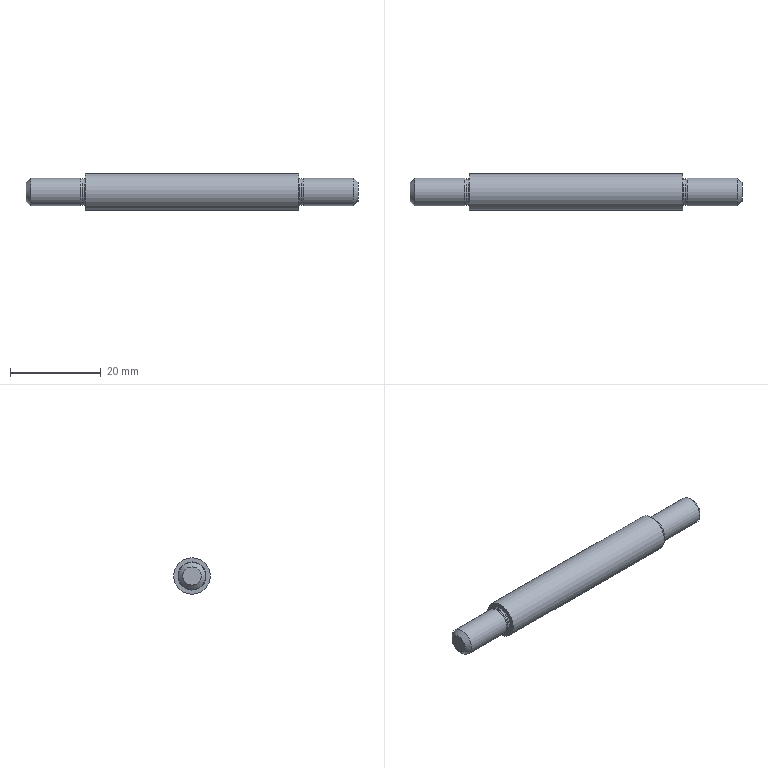Component | NX | SLIDING_GUIDE | 1 solid | 17 faces | box 73 x 8 x 8 mm | volume 3078 mm3 | cylinder 5 | plane 4 | cone 4 | torus 4 | commonest cylinder face diameters 6 x2 5.8 x2 8 x1
STEP:
#1=CARTESIAN_POINT('',(0.,0.,0.));
#2=DIRECTION('',(0.,0.,1.));
#3=DIRECTION('',(1.,0.,0.));
#4=AXIS2_PLACEMENT_3D('',#1,#2,#3);
#5=CARTESIAN_POINT('',(-36.5,15.,16.));
#6=VERTEX_POINT('',#5);
#7=CARTESIAN_POINT('',(-36.5,15.,18.));
#8=DIRECTION('',(-1.,0.,0.));
#9=DIRECTION('',(0.,0.,-1.));
#10=AXIS2_PLACEMENT_3D('',#7,#8,#9);
#11=CIRCLE('',#10,2.);
#12=CARTESIAN_POINT('',(-36.5,15.,21.));
#13=DIRECTION('',(1.,0.,0.));
#14=DIRECTION('',(0.,0.,-1.));
#15=AXIS2_PLACEMENT_3D('',#12,#13,#14);
#16=PLANE('',#15);
#17=CARTESIAN_POINT('',(5.,0.));
#18=CARTESIAN_POINT('',(5.,-3.464));
#19=CARTESIAN_POINT('',(2.,-1.732));
#20=CARTESIAN_POINT('',(-1.,-0.));
#21=CARTESIAN_POINT('',(2.,1.732));
#22=CARTESIAN_POINT('',(5.,3.464));
#23=CARTESIAN_POINT('',(5.,0.));
#24=(BOUNDED_CURVE()B_SPLINE_CURVE(2,(#17,#18,#19,#20,#21,#22,#23),.UNSPECIFIED.,.T.,.F.)B_SPLINE_CURVE_WITH_KNOTS((1,2,2,2,2,1),(-2.094,0.,2.094,4.189,6.283,8.378),.UNSPECIFIED.)CURVE()GEOMETRIC_REPRESENTATION_ITEM()RATIONAL_B_SPLINE_CURVE((1.,0.5,1.,0.5,1.,0.5,1.))REPRESENTATION_ITEM(''));
#25=(GEOMETRIC_REPRESENTATION_CONTEXT(2)PARAMETRIC_REPRESENTATION_CONTEXT()REPRESENTATION_CONTEXT('',''));
#26=DEFINITIONAL_REPRESENTATION('',(#24),#25);
#27=PCURVE('',#16,#26);
#28=CARTESIAN_POINT('',(-36.5,15.,18.));
#29=DIRECTION('',(1.,0.,0.));
#30=DIRECTION('',(0.,0.,-1.));
#31=AXIS2_PLACEMENT_3D('',#28,#29,#30);
#32=CONICAL_SURFACE('',#31,2.,0.7854);
#33=CARTESIAN_POINT('',(6.283,0.));
#34=DIRECTION('',(-1.,0.));
#35=VECTOR('',#34,1.);
#36=LINE('',#33,#35);
#37=(GEOMETRIC_REPRESENTATION_CONTEXT(2)PARAMETRIC_REPRESENTATION_CONTEXT()REPRESENTATION_CONTEXT('',''));
#38=DEFINITIONAL_REPRESENTATION('',(#36),#37);
#39=PCURVE('',#32,#38);
#40=SURFACE_CURVE('',#11,(#27,#39),.PCURVE_S1.);
#41=EDGE_CURVE('',#6,#6,#40,.T.);
#42=ORIENTED_EDGE('',*,*,#41,.T.);
#43=EDGE_LOOP('',(#42));
#44=FACE_BOUND('',#43,.T.);
#45=ADVANCED_FACE('',(#44),#16,.F.);
#46=CARTESIAN_POINT('',(-35.5,15.,15.));
#47=VERTEX_POINT('',#46);
#48=CARTESIAN_POINT('',(-35.5,15.,21.));
#49=VERTEX_POINT('',#48);
#50=CARTESIAN_POINT('',(-35.5,15.,18.));
#51=DIRECTION('',(1.,0.,0.));
#52=DIRECTION('',(0.,0.,-1.));
#53=AXIS2_PLACEMENT_3D('',#50,#51,#52);
#54=CIRCLE('',#53,3.);
#55=CARTESIAN_POINT('',(-49.5,15.,18.));
#56=DIRECTION('',(-1.,0.,0.));
#57=DIRECTION('',(0.,0.,1.));
#58=AXIS2_PLACEMENT_3D('',#55,#56,#57);
#59=CYLINDRICAL_SURFACE('',#58,3.);
#60=CARTESIAN_POINT('',(3.142,-14.));
#61=DIRECTION('',(-1.,0.));
#62=VECTOR('',#61,1.);
#63=LINE('',#60,#62);
#64=(GEOMETRIC_REPRESENTATION_CONTEXT(2)PARAMETRIC_REPRESENTATION_CONTEXT()REPRESENTATION_CONTEXT('',''));
#65=DEFINITIONAL_REPRESENTATION('',(#63),#64);
#66=PCURVE('',#59,#65);
#67=CARTESIAN_POINT('',(0.,1.));
#68=DIRECTION('',(1.,0.));
#69=VECTOR('',#68,1.);
#70=LINE('',#67,#69);
#71=(GEOMETRIC_REPRESENTATION_CONTEXT(2)PARAMETRIC_REPRESENTATION_CONTEXT()REPRESENTATION_CONTEXT('',''));
#72=DEFINITIONAL_REPRESENTATION('',(#70),#71);
#73=PCURVE('',#32,#72);
#74=SURFACE_CURVE('',#54,(#66,#73),.PCURVE_S1.);
#75=EDGE_CURVE('',#47,#49,#74,.T.);
#76=ORIENTED_EDGE('',*,*,#75,.T.);
#77=CARTESIAN_POINT('',(-24.5,15.,21.));
#78=VERTEX_POINT('',#77);
#79=CARTESIAN_POINT('',(-24.5,15.,21.));
#80=CARTESIAN_POINT('',(-35.5,15.,21.));
#81=B_SPLINE_CURVE_WITH_KNOTS('',1,(#79,#80),.UNSPECIFIED.,.F.,.F.,(2,2),(-25.,-14.),.PIECEWISE_BEZIER_KNOTS.);
#82=CARTESIAN_POINT('',(0.,0.));
#83=DIRECTION('',(0.,1.));
#84=VECTOR('',#83,1.);
#85=LINE('',#82,#84);
#86=(GEOMETRIC_REPRESENTATION_CONTEXT(2)PARAMETRIC_REPRESENTATION_CONTEXT()REPRESENTATION_CONTEXT('',''));
#87=DEFINITIONAL_REPRESENTATION('',(#85),#86);
#88=PCURVE('',#59,#87);
#89=CARTESIAN_POINT('',(6.283,0.));
#90=DIRECTION('',(0.,1.));
#91=VECTOR('',#90,1.);
#92=LINE('',#89,#91);
#93=(GEOMETRIC_REPRESENTATION_CONTEXT(2)PARAMETRIC_REPRESENTATION_CONTEXT()REPRESENTATION_CONTEXT('',''));
#94=DEFINITIONAL_REPRESENTATION('',(#92),#93);
#95=PCURVE('',#59,#94);
#96=SEAM_CURVE('',#81,(#88,#95),.PCURVE_S1.);
#97=EDGE_CURVE('',#78,#49,#96,.T.);
#98=ORIENTED_EDGE('',*,*,#97,.F.);
#99=CARTESIAN_POINT('',(-24.5,15.,18.));
#100=DIRECTION('',(-1.,0.,0.));
#101=DIRECTION('',(0.,0.,1.));
#102=AXIS2_PLACEMENT_3D('',#99,#100,#101);
#103=CIRCLE('',#102,3.);
#104=CARTESIAN_POINT('',(0.,-25.));
#105=DIRECTION('',(1.,0.));
#106=VECTOR('',#105,1.);
#107=LINE('',#104,#106);
#108=(GEOMETRIC_REPRESENTATION_CONTEXT(2)PARAMETRIC_REPRESENTATION_CONTEXT()REPRESENTATION_CONTEXT('',''));
#109=DEFINITIONAL_REPRESENTATION('',(#107),#108);
#110=PCURVE('',#59,#109);
#111=CARTESIAN_POINT('',(-24.152,15.,18.));
#112=DIRECTION('',(-1.,0.,0.));
#113=DIRECTION('',(0.,0.,1.));
#114=AXIS2_PLACEMENT_3D('',#111,#112,#113);
#115=CONICAL_SURFACE('',#114,2.907,0.2618);
#116=CARTESIAN_POINT('',(0.,0.3478));
#117=DIRECTION('',(1.,0.));
#118=VECTOR('',#117,1.);
#119=LINE('',#116,#118);
#120=(GEOMETRIC_REPRESENTATION_CONTEXT(2)PARAMETRIC_REPRESENTATION_CONTEXT()REPRESENTATION_CONTEXT('',''));
#121=DEFINITIONAL_REPRESENTATION('',(#119),#120);
#122=PCURVE('',#115,#121);
#123=SURFACE_CURVE('',#103,(#110,#122),.PCURVE_S1.);
#124=EDGE_CURVE('',#78,#78,#123,.T.);
#125=ORIENTED_EDGE('',*,*,#124,.T.);
#126=ORIENTED_EDGE('',*,*,#97,.T.);
#127=CARTESIAN_POINT('',(-35.5,15.,18.));
#128=DIRECTION('',(1.,0.,0.));
#129=DIRECTION('',(0.,0.,-1.));
#130=AXIS2_PLACEMENT_3D('',#127,#128,#129);
#131=CIRCLE('',#130,3.);
#132=CARTESIAN_POINT('',(9.425,-14.));
#133=DIRECTION('',(-1.,0.));
#134=VECTOR('',#133,1.);
#135=LINE('',#132,#134);
#136=(GEOMETRIC_REPRESENTATION_CONTEXT(2)PARAMETRIC_REPRESENTATION_CONTEXT()REPRESENTATION_CONTEXT('',''));
#137=DEFINITIONAL_REPRESENTATION('',(#135),#136);
#138=PCURVE('',#59,#137);
#139=CARTESIAN_POINT('',(0.,1.));
#140=DIRECTION('',(1.,0.));
#141=VECTOR('',#140,1.);
#142=LINE('',#139,#141);
#143=(GEOMETRIC_REPRESENTATION_CONTEXT(2)PARAMETRIC_REPRESENTATION_CONTEXT()REPRESENTATION_CONTEXT('',''));
#144=DEFINITIONAL_REPRESENTATION('',(#142),#143);
#145=PCURVE('',#32,#144);
#146=SURFACE_CURVE('',#131,(#138,#145),.PCURVE_S1.);
#147=EDGE_CURVE('',#49,#47,#146,.T.);
#148=ORIENTED_EDGE('',*,*,#147,.T.);
#149=EDGE_LOOP('',(#76,#98,#125,#126,#148));
#150=FACE_BOUND('',#149,.T.);
#151=ADVANCED_FACE('',(#150),#59,.T.);
#152=ORIENTED_EDGE('',*,*,#124,.F.);
#153=CARTESIAN_POINT('',(-24.152,15.,20.907));
#154=VERTEX_POINT('',#153);
#155=CARTESIAN_POINT('',(-24.152,15.,20.907));
#156=CARTESIAN_POINT('',(-24.5,15.,21.));
#157=B_SPLINE_CURVE_WITH_KNOTS('',1,(#155,#156),.UNSPECIFIED.,.F.,.F.,(2,2),(-0.,0.36),.PIECEWISE_BEZIER_KNOTS.);
#158=CARTESIAN_POINT('',(0.,0.));
#159=DIRECTION('',(0.,1.));
#160=VECTOR('',#159,1.);
#161=LINE('',#158,#160);
#162=(GEOMETRIC_REPRESENTATION_CONTEXT(2)PARAMETRIC_REPRESENTATION_CONTEXT()REPRESENTATION_CONTEXT('',''));
#163=DEFINITIONAL_REPRESENTATION('',(#161),#162);
#164=PCURVE('',#115,#163);
#165=CARTESIAN_POINT('',(6.283,0.));
#166=DIRECTION('',(0.,1.));
#167=VECTOR('',#166,1.);
#168=LINE('',#165,#167);
#169=(GEOMETRIC_REPRESENTATION_CONTEXT(2)PARAMETRIC_REPRESENTATION_CONTEXT()REPRESENTATION_CONTEXT('',''));
#170=DEFINITIONAL_REPRESENTATION('',(#168),#169);
#171=PCURVE('',#115,#170);
#172=SEAM_CURVE('',#157,(#164,#171),.PCURVE_S1.);
#173=EDGE_CURVE('',#154,#78,#172,.T.);
#174=ORIENTED_EDGE('',*,*,#173,.F.);
#175=CARTESIAN_POINT('',(-24.152,15.,18.));
#176=DIRECTION('',(-1.,0.,0.));
#177=DIRECTION('',(0.,0.,1.));
#178=AXIS2_PLACEMENT_3D('',#175,#176,#177);
#179=CIRCLE('',#178,2.907);
#180=CARTESIAN_POINT('',(0.,-0.));
#181=DIRECTION('',(1.,0.));
#182=VECTOR('',#181,1.);
#183=LINE('',#180,#182);
#184=(GEOMETRIC_REPRESENTATION_CONTEXT(2)PARAMETRIC_REPRESENTATION_CONTEXT()REPRESENTATION_CONTEXT('',''));
#185=DEFINITIONAL_REPRESENTATION('',(#183),#184);
#186=PCURVE('',#115,#185);
#187=CARTESIAN_POINT('',(-24.1,15.,18.));
#188=DIRECTION('',(-1.,0.,0.));
#189=DIRECTION('',(0.,0.,1.));
#190=AXIS2_PLACEMENT_3D('',#187,#188,#189);
#191=TOROIDAL_SURFACE('',#190,3.1,0.2);
#192=CARTESIAN_POINT('',(0.,9.163));
#193=DIRECTION('',(1.,0.));
#194=VECTOR('',#193,1.);
#195=LINE('',#192,#194);
#196=(GEOMETRIC_REPRESENTATION_CONTEXT(2)PARAMETRIC_REPRESENTATION_CONTEXT()REPRESENTATION_CONTEXT('',''));
#197=DEFINITIONAL_REPRESENTATION('',(#195),#196);
#198=PCURVE('',#191,#197);
#199=SURFACE_CURVE('',#179,(#186,#198),.PCURVE_S1.);
#200=EDGE_CURVE('',#154,#154,#199,.T.);
#201=ORIENTED_EDGE('',*,*,#200,.T.);
#202=ORIENTED_EDGE('',*,*,#173,.T.);
#203=EDGE_LOOP('',(#152,#174,#201,#202));
#204=FACE_BOUND('',#203,.T.);
#205=ADVANCED_FACE('',(#204),#115,.T.);
#206=ORIENTED_EDGE('',*,*,#200,.T.);
#207=CARTESIAN_POINT('',(-24.1,15.,20.9));
#208=VERTEX_POINT('',#207);
#209=CARTESIAN_POINT('',(-24.152,15.,20.907));
#210=CARTESIAN_POINT('',(-24.144,15.,20.905));
#211=CARTESIAN_POINT('',(-24.135,15.,20.903));
#212=CARTESIAN_POINT('',(-24.127,15.,20.901));
#213=CARTESIAN_POINT('',(-24.118,15.,20.9));
#214=CARTESIAN_POINT('',(-24.109,15.,20.9));
#215=CARTESIAN_POINT('',(-24.1,15.,20.9));
#216=(BOUNDED_CURVE()B_SPLINE_CURVE(6,(#209,#210,#211,#212,#213,#214,#215),.UNSPECIFIED.,.F.,.F.)B_SPLINE_CURVE_WITH_KNOTS((7,7),(2.88,3.142),.PIECEWISE_BEZIER_KNOTS.)CURVE()GEOMETRIC_REPRESENTATION_ITEM()RATIONAL_B_SPLINE_CURVE((1.001,1.,0.9999,0.9998,0.9999,1.,1.001))REPRESENTATION_ITEM(''));
#217=CARTESIAN_POINT('',(6.283,6.283));
#218=DIRECTION('',(0.,1.));
#219=VECTOR('',#218,1.);
#220=LINE('',#217,#219);
#221=(GEOMETRIC_REPRESENTATION_CONTEXT(2)PARAMETRIC_REPRESENTATION_CONTEXT()REPRESENTATION_CONTEXT('',''));
#222=DEFINITIONAL_REPRESENTATION('',(#220),#221);
#223=PCURVE('',#191,#222);
#224=CARTESIAN_POINT('',(0.,6.283));
#225=DIRECTION('',(0.,1.));
#226=VECTOR('',#225,1.);
#227=LINE('',#224,#226);
#228=(GEOMETRIC_REPRESENTATION_CONTEXT(2)PARAMETRIC_REPRESENTATION_CONTEXT()REPRESENTATION_CONTEXT('',''));
#229=DEFINITIONAL_REPRESENTATION('',(#227),#228);
#230=PCURVE('',#191,#229);
#231=SEAM_CURVE('',#216,(#223,#230),.PCURVE_S1.);
#232=EDGE_CURVE('',#154,#208,#231,.T.);
#233=ORIENTED_EDGE('',*,*,#232,.T.);
#234=CARTESIAN_POINT('',(-24.1,15.,18.));
#235=DIRECTION('',(-1.,0.,0.));
#236=DIRECTION('',(0.,0.,1.));
#237=AXIS2_PLACEMENT_3D('',#234,#235,#236);
#238=CIRCLE('',#237,2.9);
#239=CARTESIAN_POINT('',(0.,9.425));
#240=DIRECTION('',(1.,0.));
#241=VECTOR('',#240,1.);
#242=LINE('',#239,#241);
#243=(GEOMETRIC_REPRESENTATION_CONTEXT(2)PARAMETRIC_REPRESENTATION_CONTEXT()REPRESENTATION_CONTEXT('',''));
#244=DEFINITIONAL_REPRESENTATION('',(#242),#243);
#245=PCURVE('',#191,#244);
#246=CARTESIAN_POINT('',(-49.5,15.,18.));
#247=DIRECTION('',(-1.,0.,0.));
#248=DIRECTION('',(0.,0.,1.));
#249=AXIS2_PLACEMENT_3D('',#246,#247,#248);
#250=CYLINDRICAL_SURFACE('',#249,2.9);
#251=CARTESIAN_POINT('',(0.,-25.4));
#252=DIRECTION('',(1.,0.));
#253=VECTOR('',#252,1.);
#254=LINE('',#251,#253);
#255=(GEOMETRIC_REPRESENTATION_CONTEXT(2)PARAMETRIC_REPRESENTATION_CONTEXT()REPRESENTATION_CONTEXT('',''));
#256=DEFINITIONAL_REPRESENTATION('',(#254),#255);
#257=PCURVE('',#250,#256);
#258=SURFACE_CURVE('',#238,(#245,#257),.PCURVE_S1.);
#259=EDGE_CURVE('',#208,#208,#258,.T.);
#260=ORIENTED_EDGE('',*,*,#259,.F.);
#261=ORIENTED_EDGE('',*,*,#232,.F.);
#262=EDGE_LOOP('',(#206,#233,#260,#261));
#263=FACE_BOUND('',#262,.F.);
#264=ADVANCED_FACE('',(#263),#191,.F.);
#265=ORIENTED_EDGE('',*,*,#259,.F.);
#266=CARTESIAN_POINT('',(-23.7,15.,20.9));
#267=VERTEX_POINT('',#266);
#268=CARTESIAN_POINT('',(-23.7,15.,20.9));
#269=CARTESIAN_POINT('',(-24.1,15.,20.9));
#270=B_SPLINE_CURVE_WITH_KNOTS('',1,(#268,#269),.UNSPECIFIED.,.F.,.F.,(2,2),(-25.8,-25.4),.PIECEWISE_BEZIER_KNOTS.);
#271=CARTESIAN_POINT('',(0.,0.));
#272=DIRECTION('',(0.,1.));
#273=VECTOR('',#272,1.);
#274=LINE('',#271,#273);
#275=(GEOMETRIC_REPRESENTATION_CONTEXT(2)PARAMETRIC_REPRESENTATION_CONTEXT()REPRESENTATION_CONTEXT('',''));
#276=DEFINITIONAL_REPRESENTATION('',(#274),#275);
#277=PCURVE('',#250,#276);
#278=CARTESIAN_POINT('',(6.283,0.));
#279=DIRECTION('',(0.,1.));
#280=VECTOR('',#279,1.);
#281=LINE('',#278,#280);
#282=(GEOMETRIC_REPRESENTATION_CONTEXT(2)PARAMETRIC_REPRESENTATION_CONTEXT()REPRESENTATION_CONTEXT('',''));
#283=DEFINITIONAL_REPRESENTATION('',(#281),#282);
#284=PCURVE('',#250,#283);
#285=SEAM_CURVE('',#270,(#277,#284),.PCURVE_S1.);
#286=EDGE_CURVE('',#267,#208,#285,.T.);
#287=ORIENTED_EDGE('',*,*,#286,.F.);
#288=CARTESIAN_POINT('',(-23.7,15.,18.));
#289=DIRECTION('',(-1.,0.,0.));
#290=DIRECTION('',(0.,0.,1.));
#291=AXIS2_PLACEMENT_3D('',#288,#289,#290);
#292=CIRCLE('',#291,2.9);
#293=CARTESIAN_POINT('',(0.,-25.8));
#294=DIRECTION('',(1.,0.));
#295=VECTOR('',#294,1.);
#296=LINE('',#293,#295);
#297=(GEOMETRIC_REPRESENTATION_CONTEXT(2)PARAMETRIC_REPRESENTATION_CONTEXT()REPRESENTATION_CONTEXT('',''));
#298=DEFINITIONAL_REPRESENTATION('',(#296),#297);
#299=PCURVE('',#250,#298);
#300=CARTESIAN_POINT('',(-23.7,15.,18.));
#301=DIRECTION('',(-1.,0.,0.));
#302=DIRECTION('',(0.,0.,1.));
#303=AXIS2_PLACEMENT_3D('',#300,#301,#302);
#304=TOROIDAL_SURFACE('',#303,3.1,0.2);
#305=CARTESIAN_POINT('',(0.,3.142));
#306=DIRECTION('',(1.,0.));
#307=VECTOR('',#306,1.);
#308=LINE('',#305,#307);
#309=(GEOMETRIC_REPRESENTATION_CONTEXT(2)PARAMETRIC_REPRESENTATION_CONTEXT()REPRESENTATION_CONTEXT('',''));
#310=DEFINITIONAL_REPRESENTATION('',(#308),#309);
#311=PCURVE('',#304,#310);
#312=SURFACE_CURVE('',#292,(#299,#311),.PCURVE_S1.);
#313=EDGE_CURVE('',#267,#267,#312,.T.);
#314=ORIENTED_EDGE('',*,*,#313,.T.);
#315=ORIENTED_EDGE('',*,*,#286,.T.);
#316=EDGE_LOOP('',(#265,#287,#314,#315));
#317=FACE_BOUND('',#316,.T.);
#318=ADVANCED_FACE('',(#317),#250,.T.);
#319=ORIENTED_EDGE('',*,*,#313,.T.);
#320=CARTESIAN_POINT('',(-23.5,15.,21.1));
#321=VERTEX_POINT('',#320);
#322=CARTESIAN_POINT('',(-23.7,15.,20.9));
#323=CARTESIAN_POINT('',(-23.647,15.,20.9));
#324=CARTESIAN_POINT('',(-23.594,15.,20.917));
#325=CARTESIAN_POINT('',(-23.55,15.,20.95));
#326=CARTESIAN_POINT('',(-23.517,15.,20.994));
#327=CARTESIAN_POINT('',(-23.5,15.,21.047));
#328=CARTESIAN_POINT('',(-23.5,15.,21.1));
#329=(BOUNDED_CURVE()B_SPLINE_CURVE(6,(#322,#323,#324,#325,#326,#327,#328),.UNSPECIFIED.,.F.,.F.)B_SPLINE_CURVE_WITH_KNOTS((7,7),(3.142,4.712),.PIECEWISE_BEZIER_KNOTS.)CURVE()GEOMETRIC_REPRESENTATION_ITEM()RATIONAL_B_SPLINE_CURVE((1.031,1.01,0.9979,0.994,0.9979,1.01,1.031))REPRESENTATION_ITEM(''));
#330=CARTESIAN_POINT('',(6.283,0.));
#331=DIRECTION('',(0.,1.));
#332=VECTOR('',#331,1.);
#333=LINE('',#330,#332);
#334=(GEOMETRIC_REPRESENTATION_CONTEXT(2)PARAMETRIC_REPRESENTATION_CONTEXT()REPRESENTATION_CONTEXT('',''));
#335=DEFINITIONAL_REPRESENTATION('',(#333),#334);
#336=PCURVE('',#304,#335);
#337=CARTESIAN_POINT('',(0.,0.));
#338=DIRECTION('',(0.,1.));
#339=VECTOR('',#338,1.);
#340=LINE('',#337,#339);
#341=(GEOMETRIC_REPRESENTATION_CONTEXT(2)PARAMETRIC_REPRESENTATION_CONTEXT()REPRESENTATION_CONTEXT('',''));
#342=DEFINITIONAL_REPRESENTATION('',(#340),#341);
#343=PCURVE('',#304,#342);
#344=SEAM_CURVE('',#329,(#336,#343),.PCURVE_S1.);
#345=EDGE_CURVE('',#267,#321,#344,.T.);
#346=ORIENTED_EDGE('',*,*,#345,.T.);
#347=CARTESIAN_POINT('',(-23.5,15.,18.));
#348=DIRECTION('',(-1.,0.,0.));
#349=DIRECTION('',(0.,0.,1.));
#350=AXIS2_PLACEMENT_3D('',#347,#348,#349);
#351=CIRCLE('',#350,3.1);
#352=CARTESIAN_POINT('',(0.,4.712));
#353=DIRECTION('',(1.,0.));
#354=VECTOR('',#353,1.);
#355=LINE('',#352,#354);
#356=(GEOMETRIC_REPRESENTATION_CONTEXT(2)PARAMETRIC_REPRESENTATION_CONTEXT()REPRESENTATION_CONTEXT('',''));
#357=DEFINITIONAL_REPRESENTATION('',(#355),#356);
#358=PCURVE('',#304,#357);
#359=CARTESIAN_POINT('',(-23.5,15.,22.));
#360=DIRECTION('',(1.,0.,0.));
#361=DIRECTION('',(0.,0.,-1.));
#362=AXIS2_PLACEMENT_3D('',#359,#360,#361);
#363=PLANE('',#362);
#364=CARTESIAN_POINT('',(0.9,0.));
#365=CARTESIAN_POINT('',(0.9,5.369));
#366=CARTESIAN_POINT('',(5.55,2.685));
#367=CARTESIAN_POINT('',(10.2,0.));
#368=CARTESIAN_POINT('',(5.55,-2.685));
#369=CARTESIAN_POINT('',(0.9,-5.369));
#370=CARTESIAN_POINT('',(0.9,0.));
#371=(BOUNDED_CURVE()B_SPLINE_CURVE(2,(#364,#365,#366,#367,#368,#369,#370),.UNSPECIFIED.,.T.,.F.)B_SPLINE_CURVE_WITH_KNOTS((1,2,2,2,2,1),(-2.094,0.,2.094,4.189,6.283,8.378),.UNSPECIFIED.)CURVE()GEOMETRIC_REPRESENTATION_ITEM()RATIONAL_B_SPLINE_CURVE((1.,0.5,1.,0.5,1.,0.5,1.))REPRESENTATION_ITEM(''));
#372=(GEOMETRIC_REPRESENTATION_CONTEXT(2)PARAMETRIC_REPRESENTATION_CONTEXT()REPRESENTATION_CONTEXT('',''));
#373=DEFINITIONAL_REPRESENTATION('',(#371),#372);
#374=PCURVE('',#363,#373);
#375=SURFACE_CURVE('',#351,(#358,#374),.PCURVE_S1.);
#376=EDGE_CURVE('',#321,#321,#375,.T.);
#377=ORIENTED_EDGE('',*,*,#376,.F.);
#378=ORIENTED_EDGE('',*,*,#345,.F.);
#379=EDGE_LOOP('',(#319,#346,#377,#378));
#380=FACE_BOUND('',#379,.F.);
#381=ADVANCED_FACE('',(#380),#304,.F.);
#382=ORIENTED_EDGE('',*,*,#376,.F.);
#383=EDGE_LOOP('',(#382));
#384=FACE_BOUND('',#383,.T.);
#385=CARTESIAN_POINT('',(-23.5,15.,22.));
#386=VERTEX_POINT('',#385);
#387=CARTESIAN_POINT('',(-23.5,15.,18.));
#388=DIRECTION('',(-1.,0.,0.));
#389=DIRECTION('',(0.,0.,1.));
#390=AXIS2_PLACEMENT_3D('',#387,#388,#389);
#391=CIRCLE('',#390,4.);
#392=CARTESIAN_POINT('',(0.,0.));
#393=CARTESIAN_POINT('',(0.,6.928));
#394=CARTESIAN_POINT('',(6.,3.464));
#395=CARTESIAN_POINT('',(12.,0.));
#396=CARTESIAN_POINT('',(6.,-3.464));
#397=CARTESIAN_POINT('',(0.,-6.928));
#398=CARTESIAN_POINT('',(0.,0.));
#399=(BOUNDED_CURVE()B_SPLINE_CURVE(2,(#392,#393,#394,#395,#396,#397,#398),.UNSPECIFIED.,.T.,.F.)B_SPLINE_CURVE_WITH_KNOTS((1,2,2,2,2,1),(-2.094,0.,2.094,4.189,6.283,8.378),.UNSPECIFIED.)CURVE()GEOMETRIC_REPRESENTATION_ITEM()RATIONAL_B_SPLINE_CURVE((1.,0.5,1.,0.5,1.,0.5,1.))REPRESENTATION_ITEM(''));
#400=(GEOMETRIC_REPRESENTATION_CONTEXT(2)PARAMETRIC_REPRESENTATION_CONTEXT()REPRESENTATION_CONTEXT('',''));
#401=DEFINITIONAL_REPRESENTATION('',(#399),#400);
#402=PCURVE('',#363,#401);
#403=CARTESIAN_POINT('',(-49.5,15.,18.));
#404=DIRECTION('',(-1.,0.,0.));
#405=DIRECTION('',(0.,0.,1.));
#406=AXIS2_PLACEMENT_3D('',#403,#404,#405);
#407=CYLINDRICAL_SURFACE('',#406,4.);
#408=CARTESIAN_POINT('',(0.,-26.));
#409=DIRECTION('',(1.,0.));
#410=VECTOR('',#409,1.);
#411=LINE('',#408,#410);
#412=(GEOMETRIC_REPRESENTATION_CONTEXT(2)PARAMETRIC_REPRESENTATION_CONTEXT()REPRESENTATION_CONTEXT('',''));
#413=DEFINITIONAL_REPRESENTATION('',(#411),#412);
#414=PCURVE('',#407,#413);
#415=SURFACE_CURVE('',#391,(#402,#414),.PCURVE_S1.);
#416=EDGE_CURVE('',#386,#386,#415,.T.);
#417=ORIENTED_EDGE('',*,*,#416,.T.);
#418=EDGE_LOOP('',(#417));
#419=FACE_BOUND('',#418,.T.);
#420=ADVANCED_FACE('',(#384,#419),#363,.F.);
#421=ORIENTED_EDGE('',*,*,#416,.F.);
#422=CARTESIAN_POINT('',(23.5,15.,22.));
#423=VERTEX_POINT('',#422);
#424=CARTESIAN_POINT('',(23.5,15.,22.));
#425=CARTESIAN_POINT('',(-23.5,15.,22.));
#426=B_SPLINE_CURVE_WITH_KNOTS('',1,(#424,#425),.UNSPECIFIED.,.F.,.F.,(2,2),(-73.,-26.),.PIECEWISE_BEZIER_KNOTS.);
#427=CARTESIAN_POINT('',(0.,0.));
#428=DIRECTION('',(0.,1.));
#429=VECTOR('',#428,1.);
#430=LINE('',#427,#429);
#431=(GEOMETRIC_REPRESENTATION_CONTEXT(2)PARAMETRIC_REPRESENTATION_CONTEXT()REPRESENTATION_CONTEXT('',''));
#432=DEFINITIONAL_REPRESENTATION('',(#430),#431);
#433=PCURVE('',#407,#432);
#434=CARTESIAN_POINT('',(6.283,0.));
#435=DIRECTION('',(0.,1.));
#436=VECTOR('',#435,1.);
#437=LINE('',#434,#436);
#438=(GEOMETRIC_REPRESENTATION_CONTEXT(2)PARAMETRIC_REPRESENTATION_CONTEXT()REPRESENTATION_CONTEXT('',''));
#439=DEFINITIONAL_REPRESENTATION('',(#437),#438);
#440=PCURVE('',#407,#439);
#441=SEAM_CURVE('',#426,(#433,#440),.PCURVE_S1.);
#442=EDGE_CURVE('',#423,#386,#441,.T.);
#443=ORIENTED_EDGE('',*,*,#442,.F.);
#444=CARTESIAN_POINT('',(23.5,15.,18.));
#445=DIRECTION('',(-1.,0.,0.));
#446=DIRECTION('',(0.,0.,1.));
#447=AXIS2_PLACEMENT_3D('',#444,#445,#446);
#448=CIRCLE('',#447,4.);
#449=CARTESIAN_POINT('',(0.,-73.));
#450=DIRECTION('',(1.,0.));
#451=VECTOR('',#450,1.);
#452=LINE('',#449,#451);
#453=(GEOMETRIC_REPRESENTATION_CONTEXT(2)PARAMETRIC_REPRESENTATION_CONTEXT()REPRESENTATION_CONTEXT('',''));
#454=DEFINITIONAL_REPRESENTATION('',(#452),#453);
#455=PCURVE('',#407,#454);
#456=CARTESIAN_POINT('',(23.5,15.,21.1));
#457=DIRECTION('',(-1.,0.,0.));
#458=DIRECTION('',(0.,0.,1.));
#459=AXIS2_PLACEMENT_3D('',#456,#457,#458);
#460=PLANE('',#459);
#461=CARTESIAN_POINT('',(-3.1,0.));
#462=DIRECTION('',(1.,0.));
#463=AXIS2_PLACEMENT_2D('',#461,#462);
#464=CIRCLE('',#463,4.);
#465=(GEOMETRIC_REPRESENTATION_CONTEXT(2)PARAMETRIC_REPRESENTATION_CONTEXT()REPRESENTATION_CONTEXT('',''));
#466=DEFINITIONAL_REPRESENTATION('',(#464),#465);
#467=PCURVE('',#460,#466);
#468=SURFACE_CURVE('',#448,(#455,#467),.PCURVE_S1.);
#469=EDGE_CURVE('',#423,#423,#468,.T.);
#470=ORIENTED_EDGE('',*,*,#469,.T.);
#471=ORIENTED_EDGE('',*,*,#442,.T.);
#472=EDGE_LOOP('',(#421,#443,#470,#471));
#473=FACE_BOUND('',#472,.T.);
#474=ADVANCED_FACE('',(#473),#407,.T.);
#475=ORIENTED_EDGE('',*,*,#469,.F.);
#476=EDGE_LOOP('',(#475));
#477=FACE_BOUND('',#476,.T.);
#478=CARTESIAN_POINT('',(23.5,15.,21.1));
#479=VERTEX_POINT('',#478);
#480=CARTESIAN_POINT('',(23.5,15.,18.));
#481=DIRECTION('',(-1.,0.,0.));
#482=DIRECTION('',(0.,0.,1.));
#483=AXIS2_PLACEMENT_3D('',#480,#481,#482);
#484=CIRCLE('',#483,3.1);
#485=CARTESIAN_POINT('',(-3.1,0.));
#486=DIRECTION('',(1.,0.));
#487=AXIS2_PLACEMENT_2D('',#485,#486);
#488=CIRCLE('',#487,3.1);
#489=(GEOMETRIC_REPRESENTATION_CONTEXT(2)PARAMETRIC_REPRESENTATION_CONTEXT()REPRESENTATION_CONTEXT('',''));
#490=DEFINITIONAL_REPRESENTATION('',(#488),#489);
#491=PCURVE('',#460,#490);
#492=CARTESIAN_POINT('',(23.7,15.,18.));
#493=DIRECTION('',(-1.,0.,0.));
#494=DIRECTION('',(0.,0.,1.));
#495=AXIS2_PLACEMENT_3D('',#492,#493,#494);
#496=TOROIDAL_SURFACE('',#495,3.1,0.2);
#497=CARTESIAN_POINT('',(0.,7.854));
#498=DIRECTION('',(1.,0.));
#499=VECTOR('',#498,1.);
#500=LINE('',#497,#499);
#501=(GEOMETRIC_REPRESENTATION_CONTEXT(2)PARAMETRIC_REPRESENTATION_CONTEXT()REPRESENTATION_CONTEXT('',''));
#502=DEFINITIONAL_REPRESENTATION('',(#500),#501);
#503=PCURVE('',#496,#502);
#504=SURFACE_CURVE('',#484,(#491,#503),.PCURVE_S1.);
#505=EDGE_CURVE('',#479,#479,#504,.T.);
#506=ORIENTED_EDGE('',*,*,#505,.T.);
#507=EDGE_LOOP('',(#506));
#508=FACE_BOUND('',#507,.T.);
#509=ADVANCED_FACE('',(#477,#508),#460,.F.);
#510=ORIENTED_EDGE('',*,*,#505,.T.);
#511=CARTESIAN_POINT('',(23.7,15.,20.9));
#512=VERTEX_POINT('',#511);
#513=CARTESIAN_POINT('',(23.5,15.,21.1));
#514=CARTESIAN_POINT('',(23.5,15.,21.047));
#515=CARTESIAN_POINT('',(23.517,15.,20.994));
#516=CARTESIAN_POINT('',(23.55,15.,20.95));
#517=CARTESIAN_POINT('',(23.594,15.,20.917));
#518=CARTESIAN_POINT('',(23.647,15.,20.9));
#519=CARTESIAN_POINT('',(23.7,15.,20.9));
#520=(BOUNDED_CURVE()B_SPLINE_CURVE(6,(#513,#514,#515,#516,#517,#518,#519),.UNSPECIFIED.,.F.,.F.)B_SPLINE_CURVE_WITH_KNOTS((7,7),(1.571,3.142),.PIECEWISE_BEZIER_KNOTS.)CURVE()GEOMETRIC_REPRESENTATION_ITEM()RATIONAL_B_SPLINE_CURVE((1.031,1.01,0.9979,0.994,0.9979,1.01,1.031))REPRESENTATION_ITEM(''));
#521=CARTESIAN_POINT('',(6.283,6.283));
#522=DIRECTION('',(0.,1.));
#523=VECTOR('',#522,1.);
#524=LINE('',#521,#523);
#525=(GEOMETRIC_REPRESENTATION_CONTEXT(2)PARAMETRIC_REPRESENTATION_CONTEXT()REPRESENTATION_CONTEXT('',''));
#526=DEFINITIONAL_REPRESENTATION('',(#524),#525);
#527=PCURVE('',#496,#526);
#528=CARTESIAN_POINT('',(0.,6.283));
#529=DIRECTION('',(0.,1.));
#530=VECTOR('',#529,1.);
#531=LINE('',#528,#530);
#532=(GEOMETRIC_REPRESENTATION_CONTEXT(2)PARAMETRIC_REPRESENTATION_CONTEXT()REPRESENTATION_CONTEXT('',''));
#533=DEFINITIONAL_REPRESENTATION('',(#531),#532);
#534=PCURVE('',#496,#533);
#535=SEAM_CURVE('',#520,(#527,#534),.PCURVE_S1.);
#536=EDGE_CURVE('',#479,#512,#535,.T.);
#537=ORIENTED_EDGE('',*,*,#536,.T.);
#538=CARTESIAN_POINT('',(23.7,15.,18.));
#539=DIRECTION('',(-1.,0.,0.));
#540=DIRECTION('',(0.,0.,1.));
#541=AXIS2_PLACEMENT_3D('',#538,#539,#540);
#542=CIRCLE('',#541,2.9);
#543=CARTESIAN_POINT('',(0.,9.425));
#544=DIRECTION('',(1.,0.));
#545=VECTOR('',#544,1.);
#546=LINE('',#543,#545);
#547=(GEOMETRIC_REPRESENTATION_CONTEXT(2)PARAMETRIC_REPRESENTATION_CONTEXT()REPRESENTATION_CONTEXT('',''));
#548=DEFINITIONAL_REPRESENTATION('',(#546),#547);
#549=PCURVE('',#496,#548);
#550=CARTESIAN_POINT('',(-49.5,15.,18.));
#551=DIRECTION('',(-1.,0.,0.));
#552=DIRECTION('',(0.,0.,1.));
#553=AXIS2_PLACEMENT_3D('',#550,#551,#552);
#554=CYLINDRICAL_SURFACE('',#553,2.9);
#555=CARTESIAN_POINT('',(0.,-73.2));
#556=DIRECTION('',(1.,0.));
#557=VECTOR('',#556,1.);
#558=LINE('',#555,#557);
#559=(GEOMETRIC_REPRESENTATION_CONTEXT(2)PARAMETRIC_REPRESENTATION_CONTEXT()REPRESENTATION_CONTEXT('',''));
#560=DEFINITIONAL_REPRESENTATION('',(#558),#559);
#561=PCURVE('',#554,#560);
#562=SURFACE_CURVE('',#542,(#549,#561),.PCURVE_S1.);
#563=EDGE_CURVE('',#512,#512,#562,.T.);
#564=ORIENTED_EDGE('',*,*,#563,.F.);
#565=ORIENTED_EDGE('',*,*,#536,.F.);
#566=EDGE_LOOP('',(#510,#537,#564,#565));
#567=FACE_BOUND('',#566,.F.);
#568=ADVANCED_FACE('',(#567),#496,.F.);
#569=ORIENTED_EDGE('',*,*,#563,.F.);
#570=CARTESIAN_POINT('',(24.1,15.,20.9));
#571=VERTEX_POINT('',#570);
#572=CARTESIAN_POINT('',(24.1,15.,20.9));
#573=CARTESIAN_POINT('',(23.7,15.,20.9));
#574=B_SPLINE_CURVE_WITH_KNOTS('',1,(#572,#573),.UNSPECIFIED.,.F.,.F.,(2,2),(-73.6,-73.2),.PIECEWISE_BEZIER_KNOTS.);
#575=CARTESIAN_POINT('',(0.,0.));
#576=DIRECTION('',(0.,1.));
#577=VECTOR('',#576,1.);
#578=LINE('',#575,#577);
#579=(GEOMETRIC_REPRESENTATION_CONTEXT(2)PARAMETRIC_REPRESENTATION_CONTEXT()REPRESENTATION_CONTEXT('',''));
#580=DEFINITIONAL_REPRESENTATION('',(#578),#579);
#581=PCURVE('',#554,#580);
#582=CARTESIAN_POINT('',(6.283,0.));
#583=DIRECTION('',(0.,1.));
#584=VECTOR('',#583,1.);
#585=LINE('',#582,#584);
#586=(GEOMETRIC_REPRESENTATION_CONTEXT(2)PARAMETRIC_REPRESENTATION_CONTEXT()REPRESENTATION_CONTEXT('',''));
#587=DEFINITIONAL_REPRESENTATION('',(#585),#586);
#588=PCURVE('',#554,#587);
#589=SEAM_CURVE('',#574,(#581,#588),.PCURVE_S1.);
#590=EDGE_CURVE('',#571,#512,#589,.T.);
#591=ORIENTED_EDGE('',*,*,#590,.F.);
#592=CARTESIAN_POINT('',(24.1,15.,18.));
#593=DIRECTION('',(-1.,0.,0.));
#594=DIRECTION('',(0.,0.,1.));
#595=AXIS2_PLACEMENT_3D('',#592,#593,#594);
#596=CIRCLE('',#595,2.9);
#597=CARTESIAN_POINT('',(0.,-73.6));
#598=DIRECTION('',(1.,0.));
#599=VECTOR('',#598,1.);
#600=LINE('',#597,#599);
#601=(GEOMETRIC_REPRESENTATION_CONTEXT(2)PARAMETRIC_REPRESENTATION_CONTEXT()REPRESENTATION_CONTEXT('',''));
#602=DEFINITIONAL_REPRESENTATION('',(#600),#601);
#603=PCURVE('',#554,#602);
#604=CARTESIAN_POINT('',(24.1,15.,18.));
#605=DIRECTION('',(-1.,0.,0.));
#606=DIRECTION('',(0.,0.,1.));
#607=AXIS2_PLACEMENT_3D('',#604,#605,#606);
#608=TOROIDAL_SURFACE('',#607,3.1,0.2);
#609=CARTESIAN_POINT('',(0.,3.142));
#610=DIRECTION('',(1.,0.));
#611=VECTOR('',#610,1.);
#612=LINE('',#609,#611);
#613=(GEOMETRIC_REPRESENTATION_CONTEXT(2)PARAMETRIC_REPRESENTATION_CONTEXT()REPRESENTATION_CONTEXT('',''));
#614=DEFINITIONAL_REPRESENTATION('',(#612),#613);
#615=PCURVE('',#608,#614);
#616=SURFACE_CURVE('',#596,(#603,#615),.PCURVE_S1.);
#617=EDGE_CURVE('',#571,#571,#616,.T.);
#618=ORIENTED_EDGE('',*,*,#617,.T.);
#619=ORIENTED_EDGE('',*,*,#590,.T.);
#620=EDGE_LOOP('',(#569,#591,#618,#619));
#621=FACE_BOUND('',#620,.T.);
#622=ADVANCED_FACE('',(#621),#554,.T.);
#623=ORIENTED_EDGE('',*,*,#617,.T.);
#624=CARTESIAN_POINT('',(24.152,15.,20.907));
#625=VERTEX_POINT('',#624);
#626=CARTESIAN_POINT('',(24.1,15.,20.9));
#627=CARTESIAN_POINT('',(24.109,15.,20.9));
#628=CARTESIAN_POINT('',(24.118,15.,20.9));
#629=CARTESIAN_POINT('',(24.127,15.,20.901));
#630=CARTESIAN_POINT('',(24.135,15.,20.903));
#631=CARTESIAN_POINT('',(24.144,15.,20.905));
#632=CARTESIAN_POINT('',(24.152,15.,20.907));
#633=(BOUNDED_CURVE()B_SPLINE_CURVE(6,(#626,#627,#628,#629,#630,#631,#632),.UNSPECIFIED.,.F.,.F.)B_SPLINE_CURVE_WITH_KNOTS((7,7),(3.142,3.403),.PIECEWISE_BEZIER_KNOTS.)CURVE()GEOMETRIC_REPRESENTATION_ITEM()RATIONAL_B_SPLINE_CURVE((1.001,1.,0.9999,0.9998,0.9999,1.,1.001))REPRESENTATION_ITEM(''));
#634=CARTESIAN_POINT('',(6.283,0.));
#635=DIRECTION('',(0.,1.));
#636=VECTOR('',#635,1.);
#637=LINE('',#634,#636);
#638=(GEOMETRIC_REPRESENTATION_CONTEXT(2)PARAMETRIC_REPRESENTATION_CONTEXT()REPRESENTATION_CONTEXT('',''));
#639=DEFINITIONAL_REPRESENTATION('',(#637),#638);
#640=PCURVE('',#608,#639);
#641=CARTESIAN_POINT('',(0.,0.));
#642=DIRECTION('',(0.,1.));
#643=VECTOR('',#642,1.);
#644=LINE('',#641,#643);
#645=(GEOMETRIC_REPRESENTATION_CONTEXT(2)PARAMETRIC_REPRESENTATION_CONTEXT()REPRESENTATION_CONTEXT('',''));
#646=DEFINITIONAL_REPRESENTATION('',(#644),#645);
#647=PCURVE('',#608,#646);
#648=SEAM_CURVE('',#633,(#640,#647),.PCURVE_S1.);
#649=EDGE_CURVE('',#571,#625,#648,.T.);
#650=ORIENTED_EDGE('',*,*,#649,.T.);
#651=CARTESIAN_POINT('',(24.152,15.,18.));
#652=DIRECTION('',(-1.,0.,0.));
#653=DIRECTION('',(0.,0.,1.));
#654=AXIS2_PLACEMENT_3D('',#651,#652,#653);
#655=CIRCLE('',#654,2.907);
#656=CARTESIAN_POINT('',(0.,3.403));
#657=DIRECTION('',(1.,0.));
#658=VECTOR('',#657,1.);
#659=LINE('',#656,#658);
#660=(GEOMETRIC_REPRESENTATION_CONTEXT(2)PARAMETRIC_REPRESENTATION_CONTEXT()REPRESENTATION_CONTEXT('',''));
#661=DEFINITIONAL_REPRESENTATION('',(#659),#660);
#662=PCURVE('',#608,#661);
#663=CARTESIAN_POINT('',(24.5,15.,18.));
#664=DIRECTION('',(1.,0.,0.));
#665=DIRECTION('',(0.,0.,-1.));
#666=AXIS2_PLACEMENT_3D('',#663,#664,#665);
#667=CONICAL_SURFACE('',#666,3.,0.2618);
#668=CARTESIAN_POINT('',(9.425,-0.3478));
#669=DIRECTION('',(-1.,0.));
#670=VECTOR('',#669,1.);
#671=LINE('',#668,#670);
#672=(GEOMETRIC_REPRESENTATION_CONTEXT(2)PARAMETRIC_REPRESENTATION_CONTEXT()REPRESENTATION_CONTEXT('',''));
#673=DEFINITIONAL_REPRESENTATION('',(#671),#672);
#674=PCURVE('',#667,#673);
#675=SURFACE_CURVE('',#655,(#662,#674),.PCURVE_S1.);
#676=EDGE_CURVE('',#625,#625,#675,.T.);
#677=ORIENTED_EDGE('',*,*,#676,.F.);
#678=ORIENTED_EDGE('',*,*,#649,.F.);
#679=EDGE_LOOP('',(#623,#650,#677,#678));
#680=FACE_BOUND('',#679,.F.);
#681=ADVANCED_FACE('',(#680),#608,.F.);
#682=ORIENTED_EDGE('',*,*,#676,.F.);
#683=CARTESIAN_POINT('',(24.5,15.,21.));
#684=VERTEX_POINT('',#683);
#685=CARTESIAN_POINT('',(24.152,15.,20.907));
#686=CARTESIAN_POINT('',(24.5,15.,21.));
#687=B_SPLINE_CURVE_WITH_KNOTS('',1,(#685,#686),.UNSPECIFIED.,.F.,.F.,(2,2),(-0.36,0.),.PIECEWISE_BEZIER_KNOTS.);
#688=CARTESIAN_POINT('',(9.425,0.));
#689=DIRECTION('',(0.,1.));
#690=VECTOR('',#689,1.);
#691=LINE('',#688,#690);
#692=(GEOMETRIC_REPRESENTATION_CONTEXT(2)PARAMETRIC_REPRESENTATION_CONTEXT()REPRESENTATION_CONTEXT('',''));
#693=DEFINITIONAL_REPRESENTATION('',(#691),#692);
#694=PCURVE('',#667,#693);
#695=CARTESIAN_POINT('',(3.142,0.));
#696=DIRECTION('',(0.,1.));
#697=VECTOR('',#696,1.);
#698=LINE('',#695,#697);
#699=(GEOMETRIC_REPRESENTATION_CONTEXT(2)PARAMETRIC_REPRESENTATION_CONTEXT()REPRESENTATION_CONTEXT('',''));
#700=DEFINITIONAL_REPRESENTATION('',(#698),#699);
#701=PCURVE('',#667,#700);
#702=SEAM_CURVE('',#687,(#694,#701),.PCURVE_S1.);
#703=EDGE_CURVE('',#625,#684,#702,.T.);
#704=ORIENTED_EDGE('',*,*,#703,.T.);
#705=CARTESIAN_POINT('',(24.5,15.,18.));
#706=DIRECTION('',(-1.,0.,0.));
#707=DIRECTION('',(0.,0.,1.));
#708=AXIS2_PLACEMENT_3D('',#705,#706,#707);
#709=CIRCLE('',#708,3.);
#710=CARTESIAN_POINT('',(9.425,0.));
#711=DIRECTION('',(-1.,0.));
#712=VECTOR('',#711,1.);
#713=LINE('',#710,#712);
#714=(GEOMETRIC_REPRESENTATION_CONTEXT(2)PARAMETRIC_REPRESENTATION_CONTEXT()REPRESENTATION_CONTEXT('',''));
#715=DEFINITIONAL_REPRESENTATION('',(#713),#714);
#716=PCURVE('',#667,#715);
#717=CARTESIAN_POINT('',(-49.5,15.,18.));
#718=DIRECTION('',(-1.,0.,0.));
#719=DIRECTION('',(0.,0.,1.));
#720=AXIS2_PLACEMENT_3D('',#717,#718,#719);
#721=CYLINDRICAL_SURFACE('',#720,3.);
#722=CARTESIAN_POINT('',(0.,-74.));
#723=DIRECTION('',(1.,0.));
#724=VECTOR('',#723,1.);
#725=LINE('',#722,#724);
#726=(GEOMETRIC_REPRESENTATION_CONTEXT(2)PARAMETRIC_REPRESENTATION_CONTEXT()REPRESENTATION_CONTEXT('',''));
#727=DEFINITIONAL_REPRESENTATION('',(#725),#726);
#728=PCURVE('',#721,#727);
#729=SURFACE_CURVE('',#709,(#716,#728),.PCURVE_S1.);
#730=EDGE_CURVE('',#684,#684,#729,.T.);
#731=ORIENTED_EDGE('',*,*,#730,.T.);
#732=ORIENTED_EDGE('',*,*,#703,.F.);
#733=EDGE_LOOP('',(#682,#704,#731,#732));
#734=FACE_BOUND('',#733,.T.);
#735=ADVANCED_FACE('',(#734),#667,.T.);
#736=CARTESIAN_POINT('',(35.5,15.,21.));
#737=VERTEX_POINT('',#736);
#738=CARTESIAN_POINT('',(35.5,15.,18.));
#739=DIRECTION('',(-1.,0.,0.));
#740=DIRECTION('',(0.,0.,1.));
#741=AXIS2_PLACEMENT_3D('',#738,#739,#740);
#742=CIRCLE('',#741,3.);
#743=CARTESIAN_POINT('',(0.,-85.));
#744=DIRECTION('',(1.,0.));
#745=VECTOR('',#744,1.);
#746=LINE('',#743,#745);
#747=(GEOMETRIC_REPRESENTATION_CONTEXT(2)PARAMETRIC_REPRESENTATION_CONTEXT()REPRESENTATION_CONTEXT('',''));
#748=DEFINITIONAL_REPRESENTATION('',(#746),#747);
#749=PCURVE('',#721,#748);
#750=CARTESIAN_POINT('',(35.5,15.,18.));
#751=DIRECTION('',(-1.,0.,0.));
#752=DIRECTION('',(0.,0.,1.));
#753=AXIS2_PLACEMENT_3D('',#750,#751,#752);
#754=CONICAL_SURFACE('',#753,3.,0.7854);
#755=CARTESIAN_POINT('',(0.,0.));
#756=DIRECTION('',(1.,0.));
#757=VECTOR('',#756,1.);
#758=LINE('',#755,#757);
#759=(GEOMETRIC_REPRESENTATION_CONTEXT(2)PARAMETRIC_REPRESENTATION_CONTEXT()REPRESENTATION_CONTEXT('',''));
#760=DEFINITIONAL_REPRESENTATION('',(#758),#759);
#761=PCURVE('',#754,#760);
#762=SURFACE_CURVE('',#742,(#749,#761),.PCURVE_S1.);
#763=EDGE_CURVE('',#737,#737,#762,.T.);
#764=ORIENTED_EDGE('',*,*,#763,.T.);
#765=CARTESIAN_POINT('',(35.5,15.,21.));
#766=CARTESIAN_POINT('',(24.5,15.,21.));
#767=B_SPLINE_CURVE_WITH_KNOTS('',1,(#765,#766),.UNSPECIFIED.,.F.,.F.,(2,2),(-85.,-74.),.PIECEWISE_BEZIER_KNOTS.);
#768=CARTESIAN_POINT('',(6.283,0.));
#769=DIRECTION('',(0.,1.));
#770=VECTOR('',#769,1.);
#771=LINE('',#768,#770);
#772=(GEOMETRIC_REPRESENTATION_CONTEXT(2)PARAMETRIC_REPRESENTATION_CONTEXT()REPRESENTATION_CONTEXT('',''));
#773=DEFINITIONAL_REPRESENTATION('',(#771),#772);
#774=PCURVE('',#721,#773);
#775=CARTESIAN_POINT('',(0.,0.));
#776=DIRECTION('',(0.,1.));
#777=VECTOR('',#776,1.);
#778=LINE('',#775,#777);
#779=(GEOMETRIC_REPRESENTATION_CONTEXT(2)PARAMETRIC_REPRESENTATION_CONTEXT()REPRESENTATION_CONTEXT('',''));
#780=DEFINITIONAL_REPRESENTATION('',(#778),#779);
#781=PCURVE('',#721,#780);
#782=SEAM_CURVE('',#767,(#774,#781),.PCURVE_S1.);
#783=EDGE_CURVE('',#737,#684,#782,.T.);
#784=ORIENTED_EDGE('',*,*,#783,.T.);
#785=ORIENTED_EDGE('',*,*,#730,.F.);
#786=ORIENTED_EDGE('',*,*,#783,.F.);
#787=EDGE_LOOP('',(#764,#784,#785,#786));
#788=FACE_BOUND('',#787,.T.);
#789=ADVANCED_FACE('',(#788),#721,.T.);
#790=CARTESIAN_POINT('',(36.5,15.,20.));
#791=VERTEX_POINT('',#790);
#792=CARTESIAN_POINT('',(36.5,15.,18.));
#793=DIRECTION('',(1.,0.,0.));
#794=DIRECTION('',(0.,0.,1.));
#795=AXIS2_PLACEMENT_3D('',#792,#793,#794);
#796=CIRCLE('',#795,2.);
#797=CARTESIAN_POINT('',(36.5,15.,18.));
#798=DIRECTION('',(-1.,0.,0.));
#799=DIRECTION('',(0.,0.,1.));
#800=AXIS2_PLACEMENT_3D('',#797,#798,#799);
#801=PLANE('',#800);
#802=CARTESIAN_POINT('',(2.,0.));
#803=CARTESIAN_POINT('',(2.,-3.464));
#804=CARTESIAN_POINT('',(-1.,-1.732));
#805=CARTESIAN_POINT('',(-4.,-0.));
#806=CARTESIAN_POINT('',(-1.,1.732));
#807=CARTESIAN_POINT('',(2.,3.464));
#808=CARTESIAN_POINT('',(2.,0.));
#809=(BOUNDED_CURVE()B_SPLINE_CURVE(2,(#802,#803,#804,#805,#806,#807,#808),.UNSPECIFIED.,.T.,.F.)B_SPLINE_CURVE_WITH_KNOTS((1,2,2,2,2,1),(-2.094,0.,2.094,4.189,6.283,8.378),.UNSPECIFIED.)CURVE()GEOMETRIC_REPRESENTATION_ITEM()RATIONAL_B_SPLINE_CURVE((1.,0.5,1.,0.5,1.,0.5,1.))REPRESENTATION_ITEM(''));
#810=(GEOMETRIC_REPRESENTATION_CONTEXT(2)PARAMETRIC_REPRESENTATION_CONTEXT()REPRESENTATION_CONTEXT('',''));
#811=DEFINITIONAL_REPRESENTATION('',(#809),#810);
#812=PCURVE('',#801,#811);
#813=CARTESIAN_POINT('',(6.283,-1.));
#814=DIRECTION('',(-1.,0.));
#815=VECTOR('',#814,1.);
#816=LINE('',#813,#815);
#817=(GEOMETRIC_REPRESENTATION_CONTEXT(2)PARAMETRIC_REPRESENTATION_CONTEXT()REPRESENTATION_CONTEXT('',''));
#818=DEFINITIONAL_REPRESENTATION('',(#816),#817);
#819=PCURVE('',#754,#818);
#820=SURFACE_CURVE('',#796,(#812,#819),.PCURVE_S1.);
#821=EDGE_CURVE('',#791,#791,#820,.T.);
#822=ORIENTED_EDGE('',*,*,#821,.T.);
#823=EDGE_LOOP('',(#822));
#824=FACE_BOUND('',#823,.T.);
#825=ADVANCED_FACE('',(#824),#801,.F.);
#826=ORIENTED_EDGE('',*,*,#75,.F.);
#827=CARTESIAN_POINT('',(-36.5,15.,16.));
#828=CARTESIAN_POINT('',(-35.5,15.,15.));
#829=B_SPLINE_CURVE_WITH_KNOTS('',1,(#827,#828),.UNSPECIFIED.,.F.,.F.,(2,2),(0.,1.414),.PIECEWISE_BEZIER_KNOTS.);
#830=CARTESIAN_POINT('',(0.,0.));
#831=DIRECTION('',(0.,1.));
#832=VECTOR('',#831,1.);
#833=LINE('',#830,#832);
#834=(GEOMETRIC_REPRESENTATION_CONTEXT(2)PARAMETRIC_REPRESENTATION_CONTEXT()REPRESENTATION_CONTEXT('',''));
#835=DEFINITIONAL_REPRESENTATION('',(#833),#834);
#836=PCURVE('',#32,#835);
#837=CARTESIAN_POINT('',(6.283,0.));
#838=DIRECTION('',(0.,1.));
#839=VECTOR('',#838,1.);
#840=LINE('',#837,#839);
#841=(GEOMETRIC_REPRESENTATION_CONTEXT(2)PARAMETRIC_REPRESENTATION_CONTEXT()REPRESENTATION_CONTEXT('',''));
#842=DEFINITIONAL_REPRESENTATION('',(#840),#841);
#843=PCURVE('',#32,#842);
#844=SEAM_CURVE('',#829,(#836,#843),.PCURVE_S1.);
#845=EDGE_CURVE('',#6,#47,#844,.T.);
#846=ORIENTED_EDGE('',*,*,#845,.F.);
#847=ORIENTED_EDGE('',*,*,#41,.F.);
#848=ORIENTED_EDGE('',*,*,#845,.T.);
#849=ORIENTED_EDGE('',*,*,#147,.F.);
#850=EDGE_LOOP('',(#826,#846,#847,#848,#849));
#851=FACE_BOUND('',#850,.T.);
#852=ADVANCED_FACE('',(#851),#32,.T.);
#853=ORIENTED_EDGE('',*,*,#821,.F.);
#854=CARTESIAN_POINT('',(36.5,15.,20.));
#855=CARTESIAN_POINT('',(35.5,15.,21.));
#856=B_SPLINE_CURVE_WITH_KNOTS('',1,(#854,#855),.UNSPECIFIED.,.F.,.F.,(2,2),(-1.414,0.),.PIECEWISE_BEZIER_KNOTS.);
#857=CARTESIAN_POINT('',(6.283,0.));
#858=DIRECTION('',(0.,1.));
#859=VECTOR('',#858,1.);
#860=LINE('',#857,#859);
#861=(GEOMETRIC_REPRESENTATION_CONTEXT(2)PARAMETRIC_REPRESENTATION_CONTEXT()REPRESENTATION_CONTEXT('',''));
#862=DEFINITIONAL_REPRESENTATION('',(#860),#861);
#863=PCURVE('',#754,#862);
#864=CARTESIAN_POINT('',(0.,0.));
#865=DIRECTION('',(0.,1.));
#866=VECTOR('',#865,1.);
#867=LINE('',#864,#866);
#868=(GEOMETRIC_REPRESENTATION_CONTEXT(2)PARAMETRIC_REPRESENTATION_CONTEXT()REPRESENTATION_CONTEXT('',''));
#869=DEFINITIONAL_REPRESENTATION('',(#867),#868);
#870=PCURVE('',#754,#869);
#871=SEAM_CURVE('',#856,(#863,#870),.PCURVE_S1.);
#872=EDGE_CURVE('',#791,#737,#871,.T.);
#873=ORIENTED_EDGE('',*,*,#872,.T.);
#874=ORIENTED_EDGE('',*,*,#763,.F.);
#875=ORIENTED_EDGE('',*,*,#872,.F.);
#876=EDGE_LOOP('',(#853,#873,#874,#875));
#877=FACE_BOUND('',#876,.T.);
#878=ADVANCED_FACE('',(#877),#754,.T.);
#879=CLOSED_SHELL('',(#45,#151,#205,#264,#318,#381,#420,#474,#509,#568,#622,#681,#735,#789,#825,#852,#878));
#880=MANIFOLD_SOLID_BREP('',#879);
#881=(LENGTH_UNIT()NAMED_UNIT(*)SI_UNIT(.MILLI.,.METRE.));
#882=UNCERTAINTY_MEASURE_WITH_UNIT(LENGTH_MEASURE(0.00001),#881,'','');
#883=(NAMED_UNIT(*)PLANE_ANGLE_UNIT()SI_UNIT($,.RADIAN.));
#884=(NAMED_UNIT(*)SI_UNIT($,.STERADIAN.)SOLID_ANGLE_UNIT());
#885=(GEOMETRIC_REPRESENTATION_CONTEXT(3)GLOBAL_UNCERTAINTY_ASSIGNED_CONTEXT((#882))GLOBAL_UNIT_ASSIGNED_CONTEXT((#881,#883,#884))REPRESENTATION_CONTEXT('',''));
#886=ADVANCED_BREP_SHAPE_REPRESENTATION('',(#4,#880),#885);